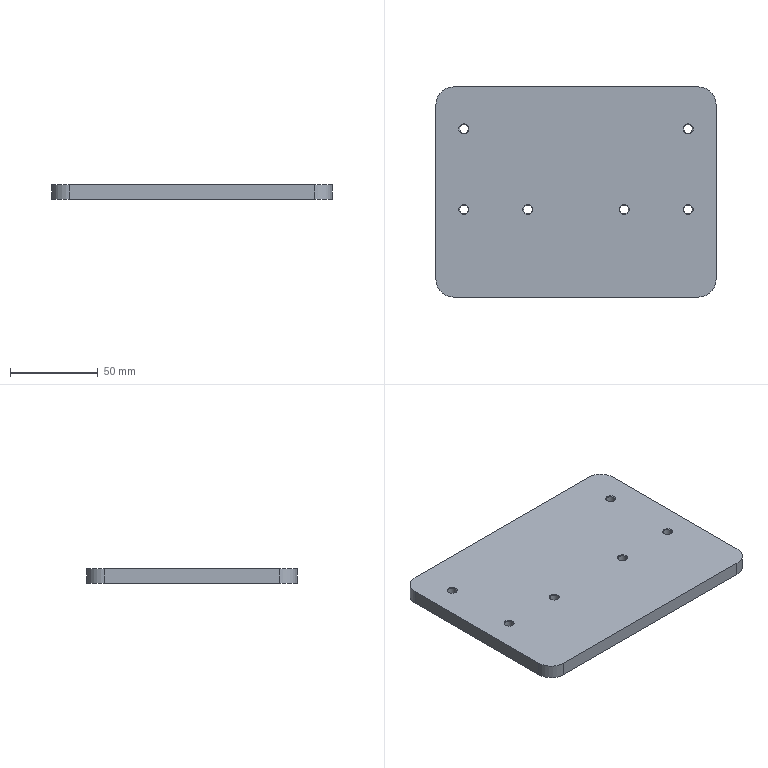Component | NX | BASE | 1 solid | 28 faces | volume 151955 mm3 | cone 12 | cylinder 10 | plane 6 | commonest cylinder face diameters 5 x6 20 x4